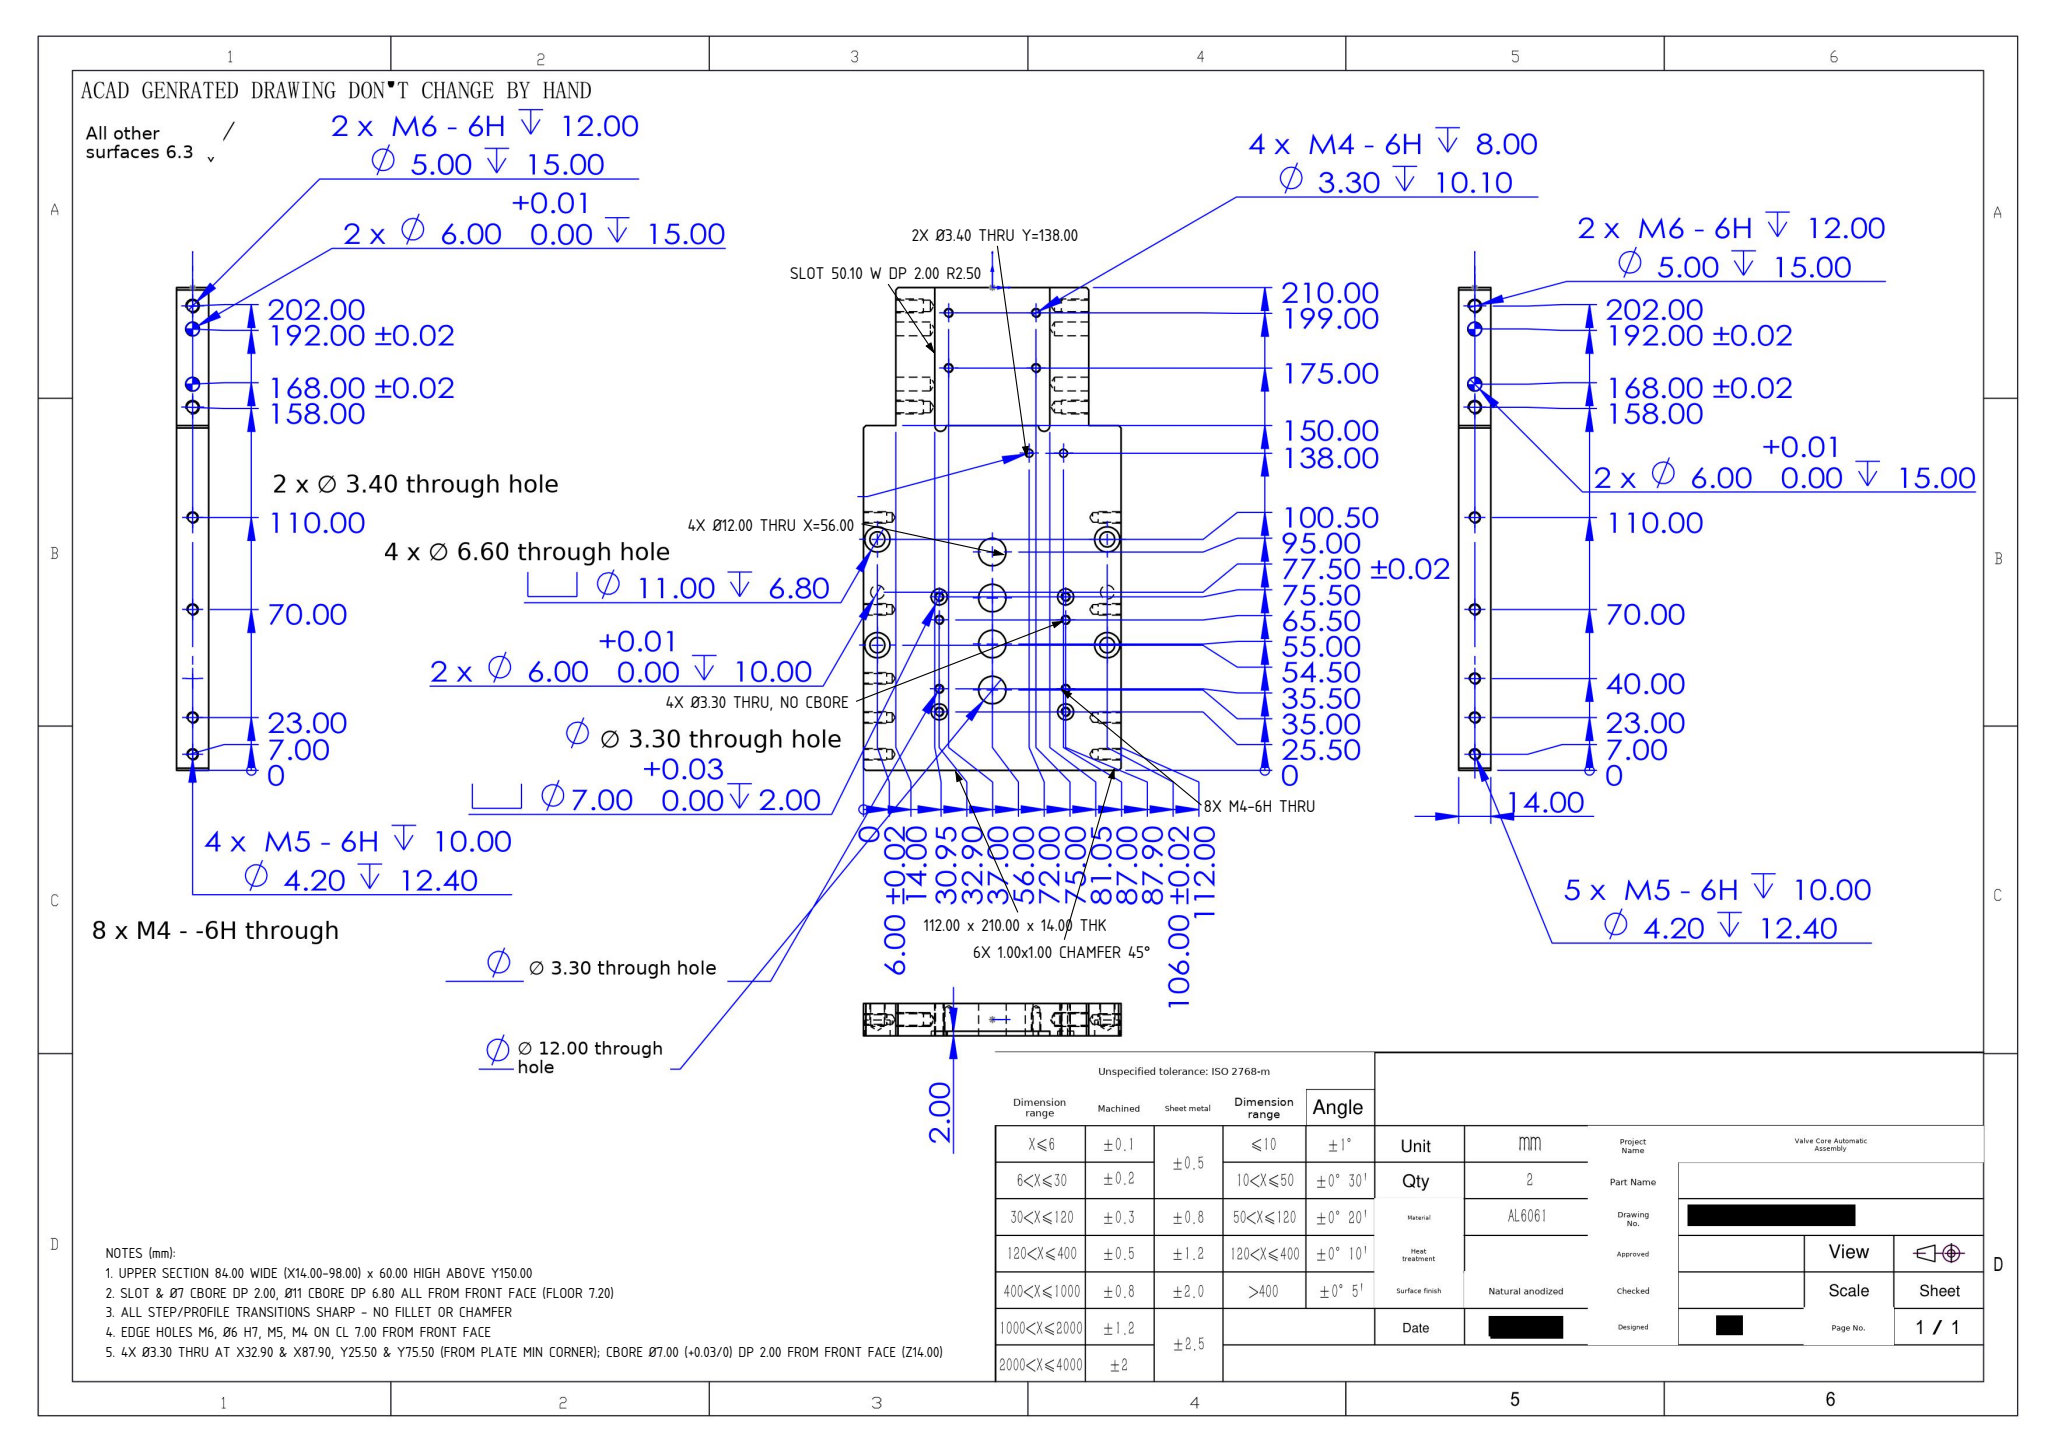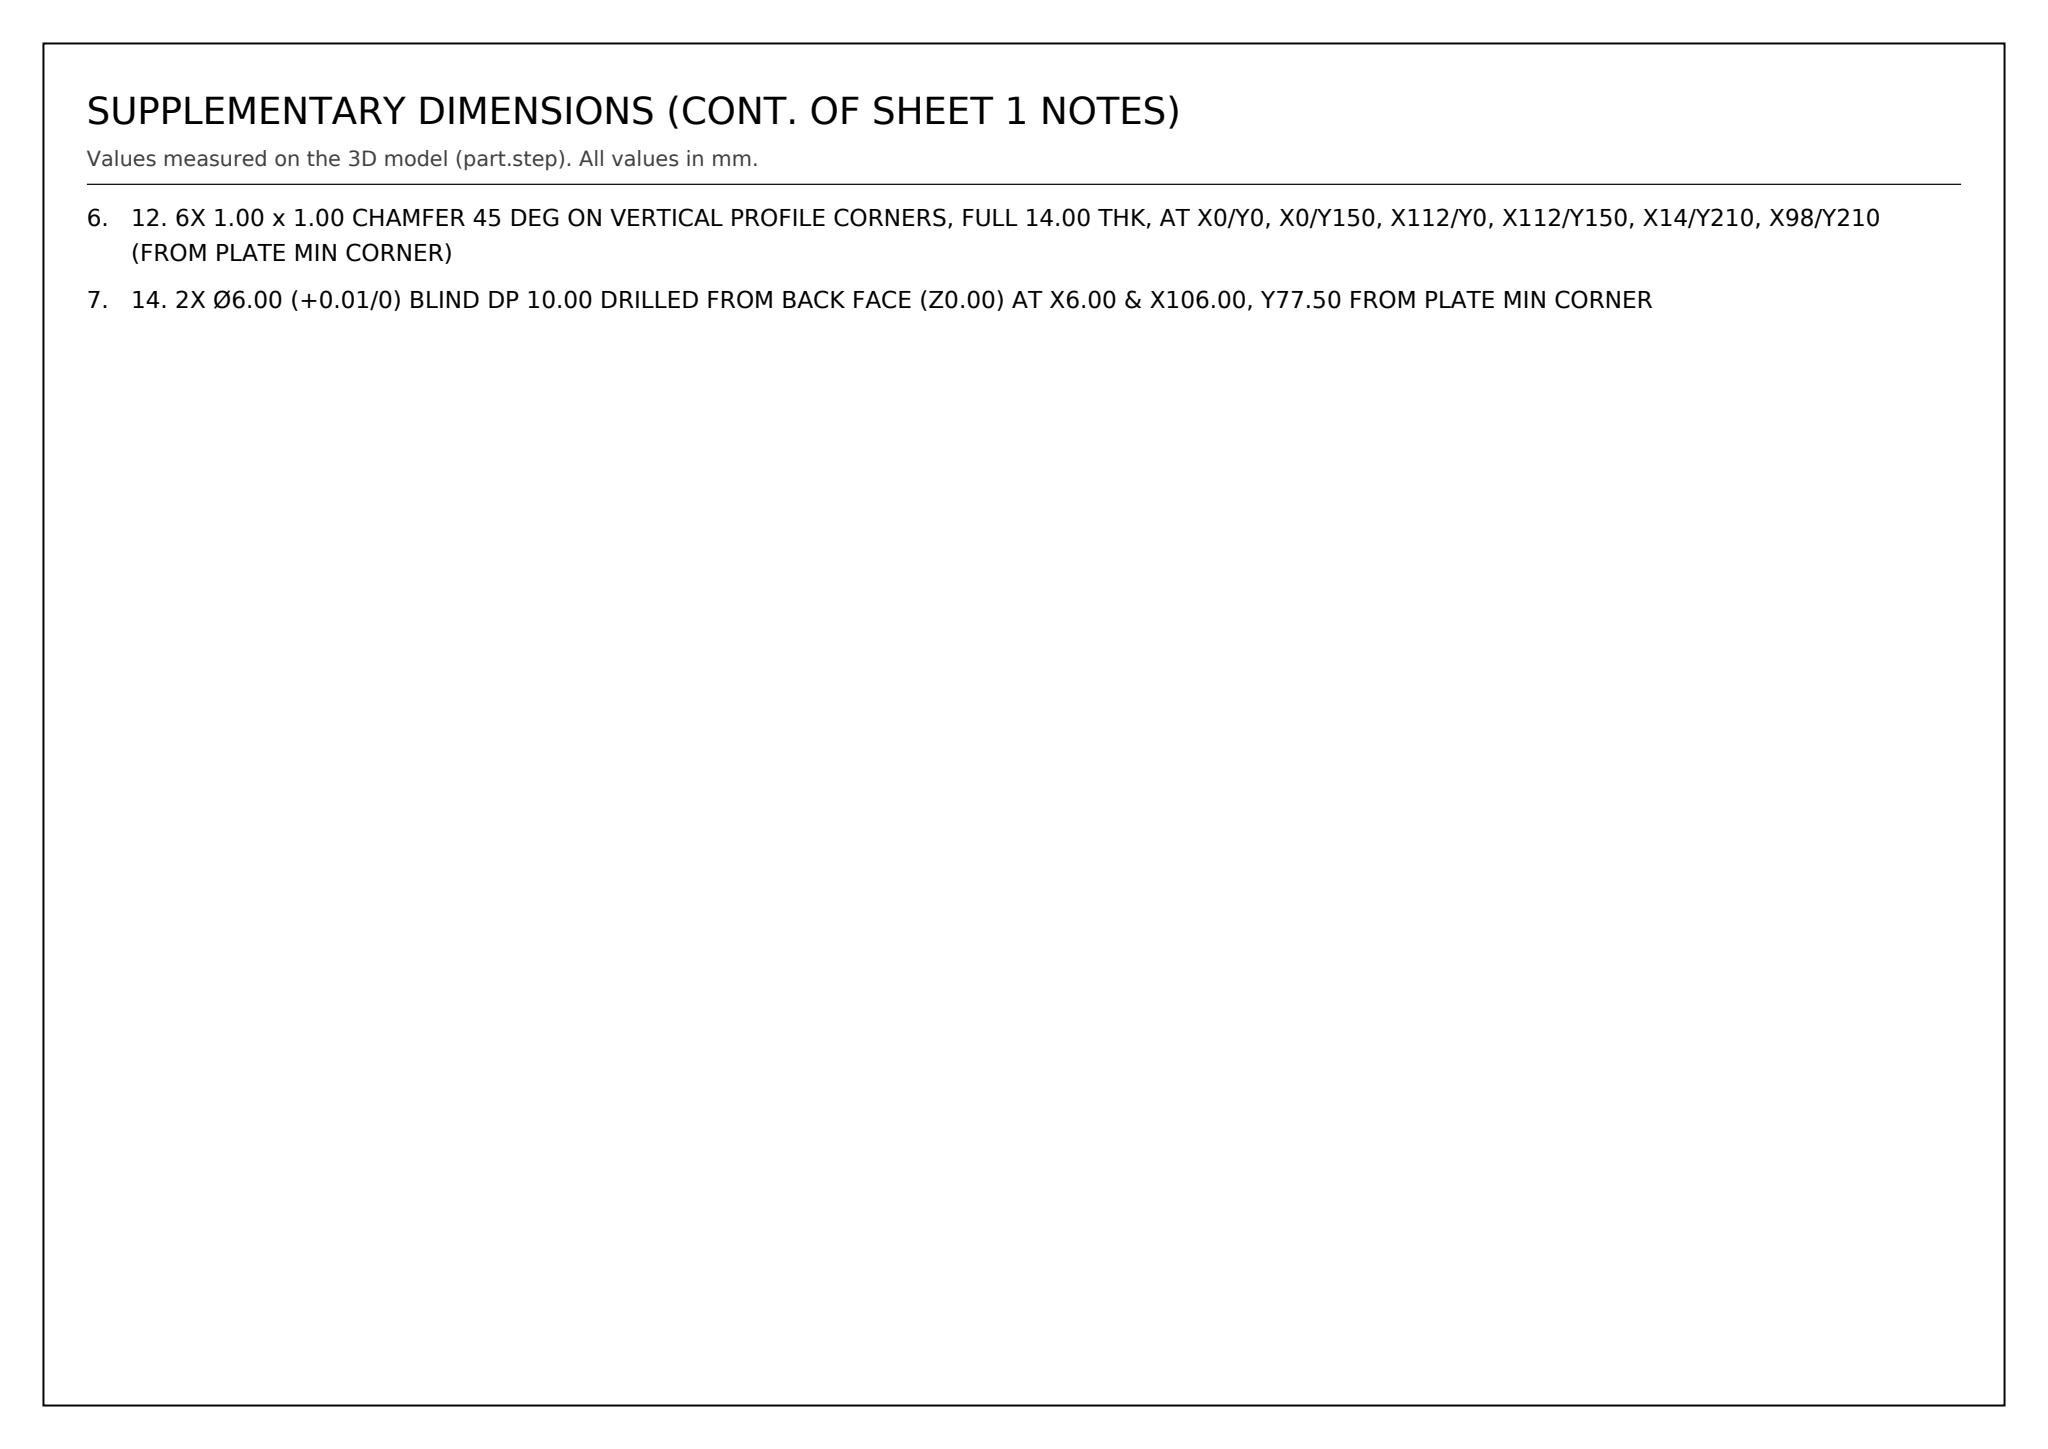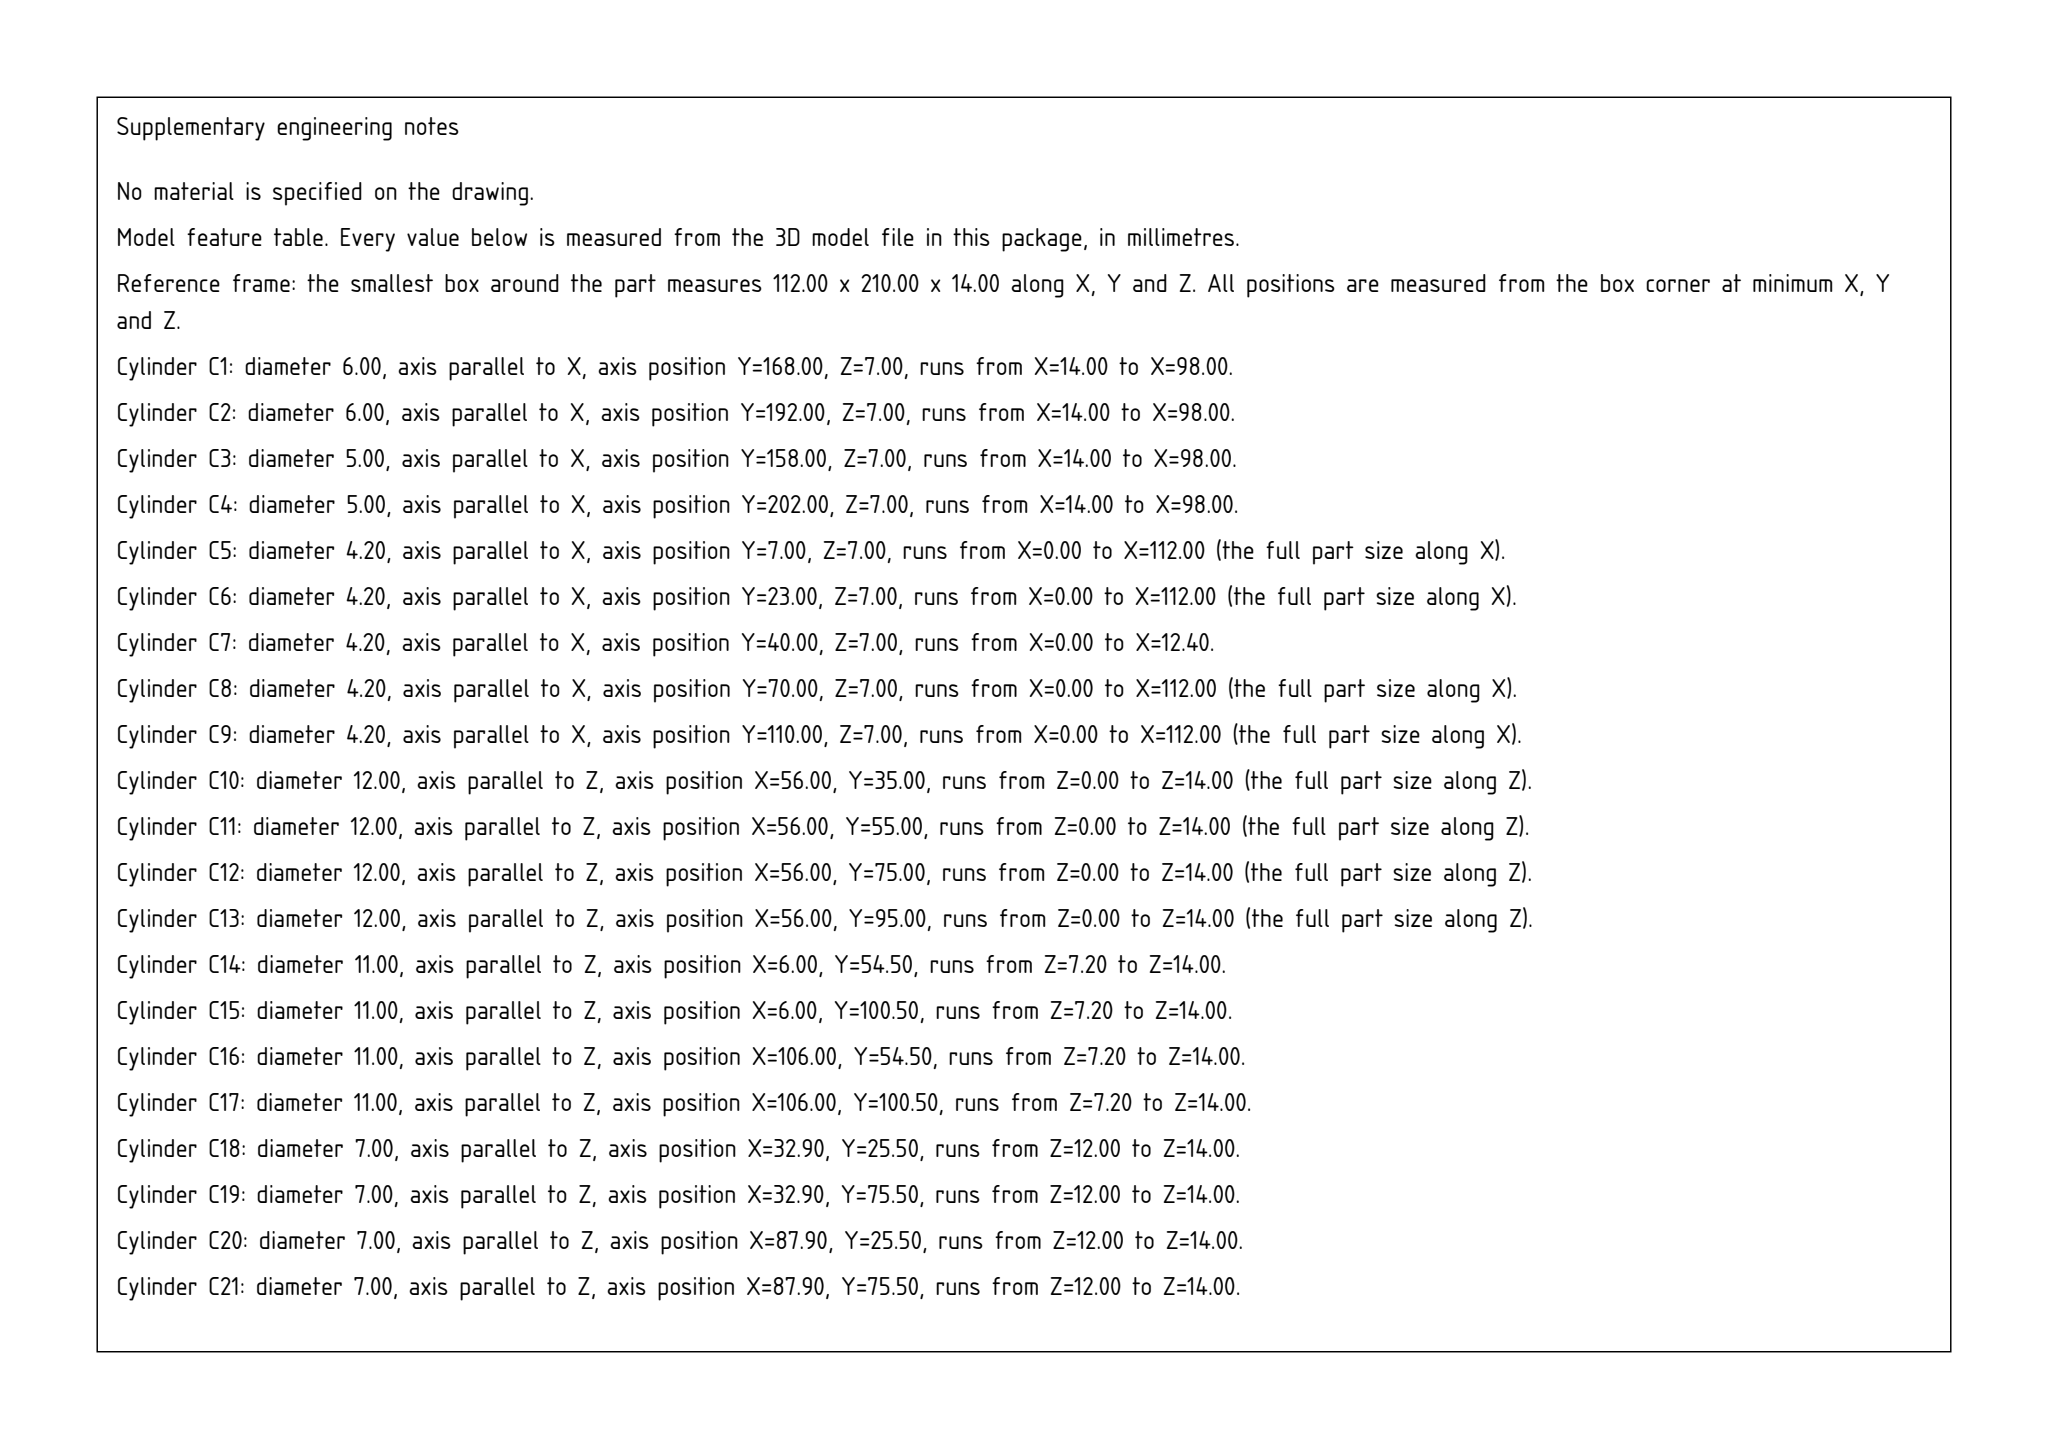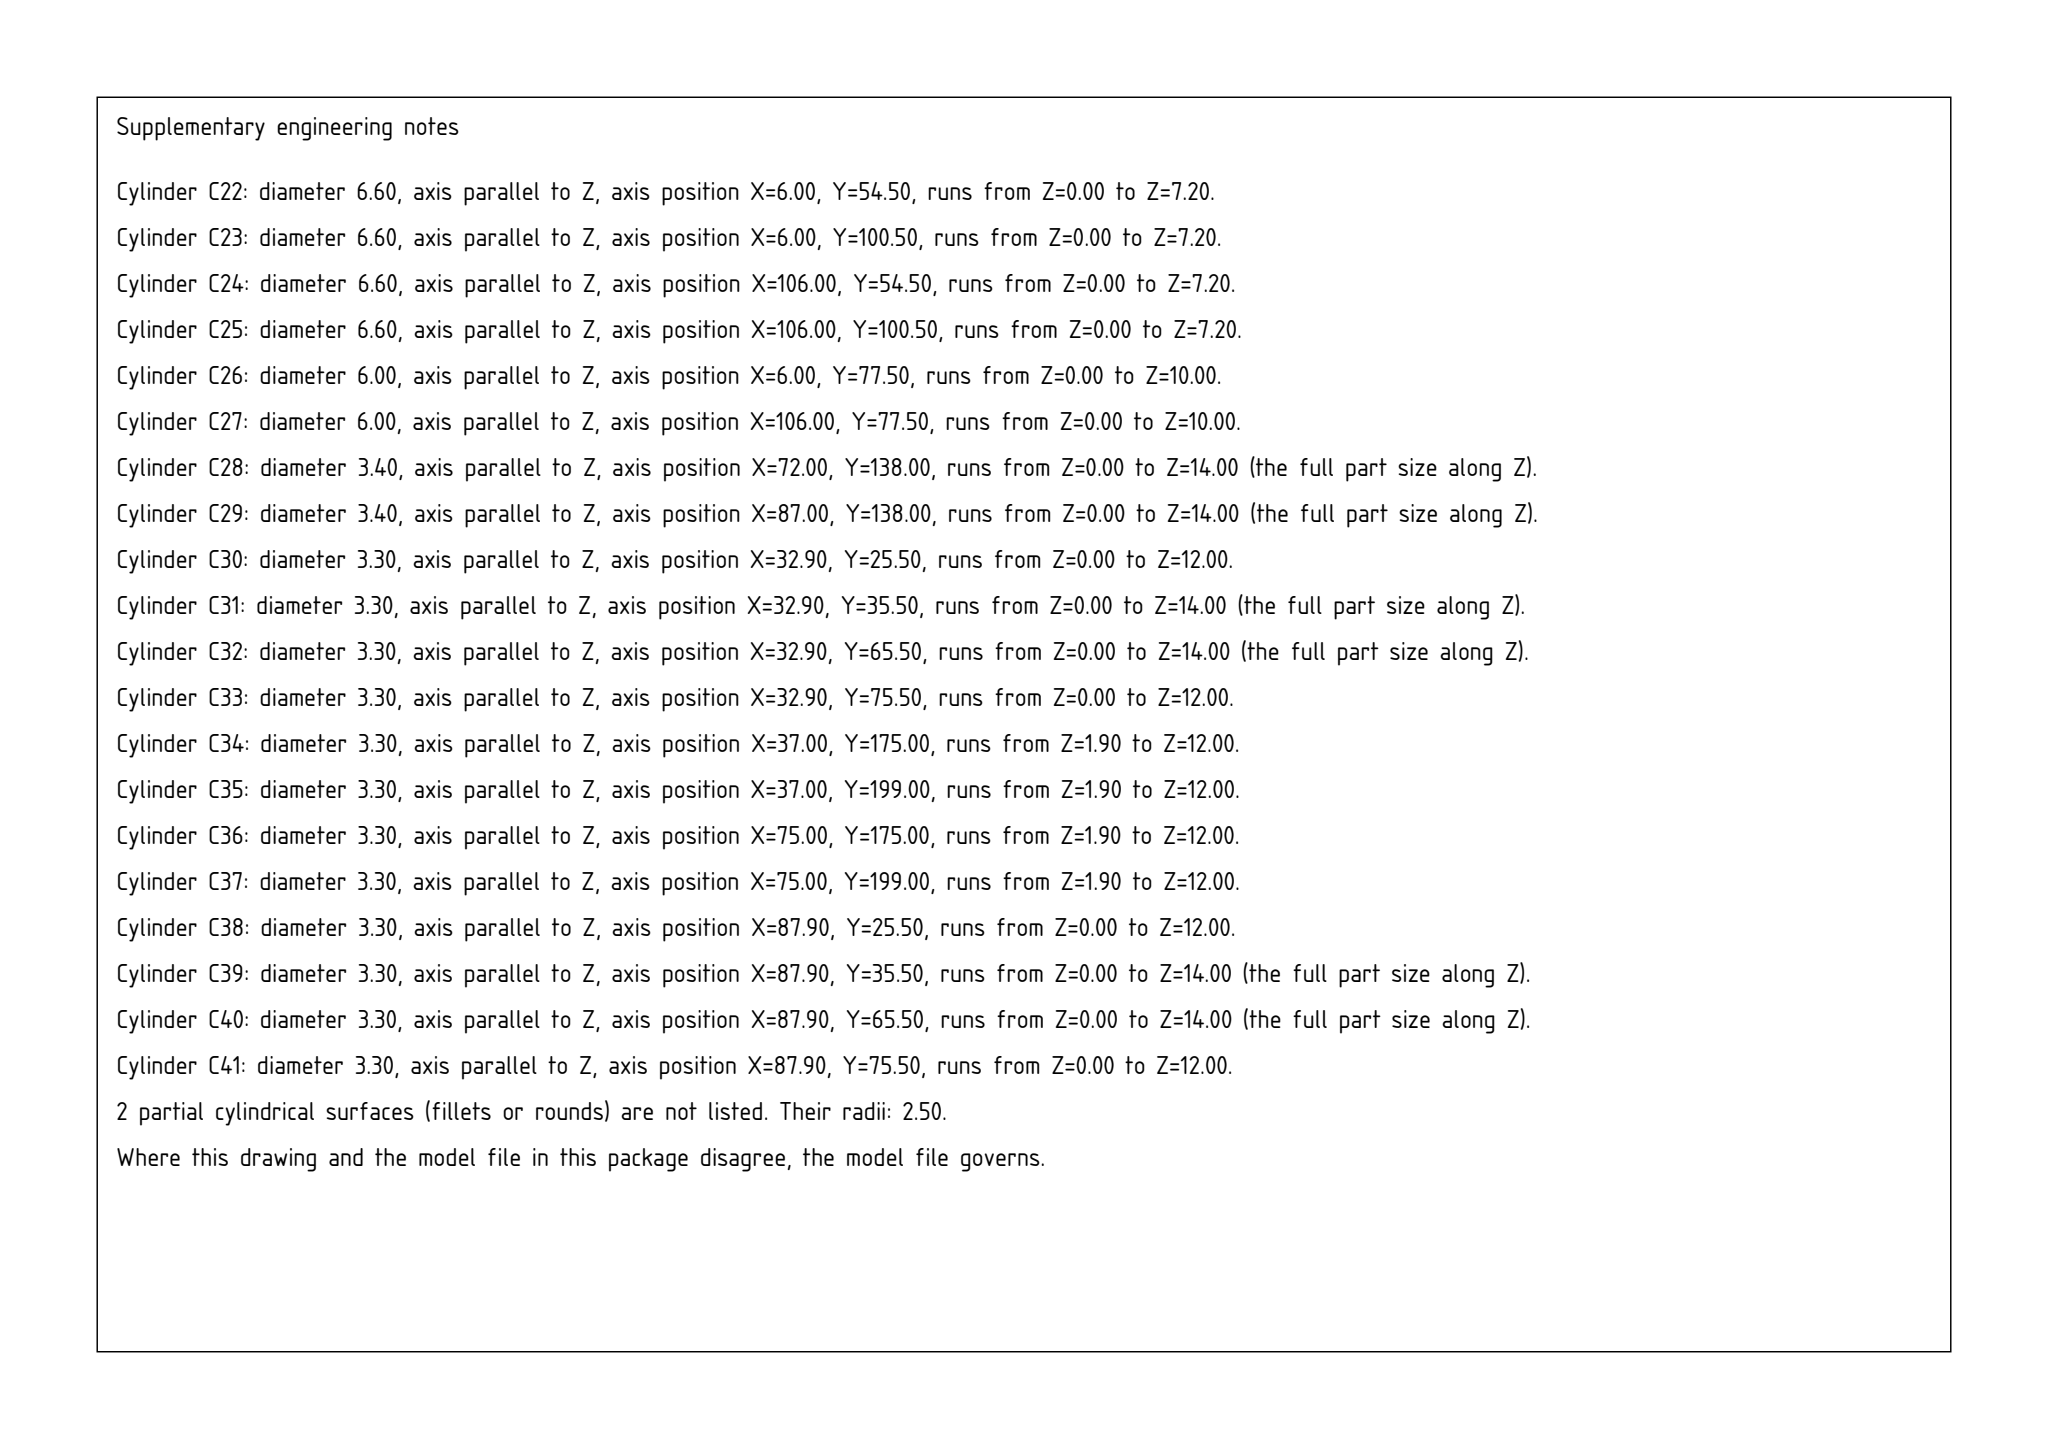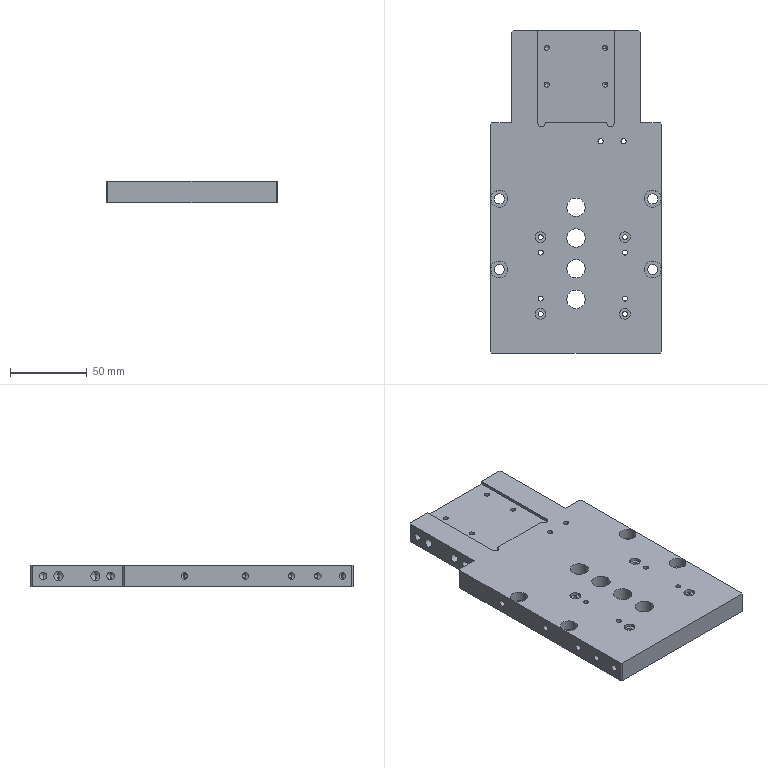Part | SolidWorks | mm | material AL6061 | 1 solid | 174 faces | box 112 x 210 x 14 mm | volume 282775 mm3 | cylinder 100 | cone 46 | plane 28 | commonest cylinder face diameters 3.3 x24 4.2 x18 6 x12 5 x10 7 x8 11 x8 6.6 x8 12 x8
Drawing notes:
PLATE 112.00 x 210.00 x 14.00 THK; UNIFORM, NO STEPS IN Z | from the solid: bbox 112x210, bbox_z=14.0; only full z faces at 0.0 and 14.0
UPPER SECTION 84.00 WIDE (X14.00-98.00) x 60.00 HIGH ABOVE Y150.00 | from the solid: X planes 14.0 & 98.0 bound upper section; Y 150.0 step to 210.0 top
SLOT 50.10 WIDE (X30.95-81.05) OPEN AT TOP, DP 2.00, END Y150.00, R2.50 CNRS | from the solid: X planes 30.95/81.05; floor z=12.0 (14.0-2.0); open face at y=210; Ø5 z-cyls at (33.45,150) & (78.55,150) len 2.0; 3 faces at y=150
SLOT & Ø7 CBORE DP 2.00, Ø11 CBORE DP 6.80 ALL FROM FRONT FACE (FLOOR 7.20) | from the solid: z planes 12.0 (slot floor + 4x Ø7 cbore) and 7.2 (4x Ø11 cbore = 14.0-6.8)
ALL STEP/PROFILE TRANSITIONS SHARP - NO FILLET OR CHAMFER | from the solid: fillet_radii empty; no cones except 118° drill points
4 x Ø12.00 THRU AT X56.00; Y35.00, 55.00, 75.00, 95.00 | from the solid: Ø12 z-cyls len 14.0 at (56,35), (56,55), (56,75), (56,95)
2 x Ø3.40 THRU AT Y138.00; X72.00 & 87.00 | from the solid: Ø3.4 z-cyls at (72.0,138.0) and (87.0,138.0), length 14.0 = full thk
8 x M4-6H THRU AT X32.90 & 87.90; Y25.50, 35.50, 65.50, 75.50 | from the solid: Ø3.30 z-holes at x=32.9 & 87.9, y=25.5/35.5/65.5/75.5, thru 14.0 or 12.0 under Ø7 CBORE
EDGE HOLES M6, Ø6 H7, M5, M4 ON CL 7.00 FROM FRONT FACE | from the solid: x-axis cylinders Ø4.2/5.0/6.0 all at z=7.0 of 14.0 thk plate
4X Ø3.30 THRU AT X32.90 & X87.90, Y25.50 & Y75.50 (FROM PLATE MIN CORNER); CBORE Ø7.00 (+0.03/0) DP 2.00 FROM FRONT FACE (Z14.00) | from the solid: cylinders: Ø3.3 z-holes at (32.9,25.5),(32.9,75.5),(87.9,25.5),(87.9,75.5) from 0.0 to 12.0, each with Ø7.0 z-bore from 12.0 to 14.0
4X Ø3.30 THRU (NO CBORE) AT X32.90 & X87.90, Y35.50 & Y65.50 FROM PLATE MIN CORNER | from the solid: cylinders: Ø3.3 z-holes at (32.9,35.5),(32.9,65.5),(87.9,35.5),(87.9,65.5) from 0.0 to 14.0
12. 6X 1.00 x 1.00 CHAMFER 45 DEG ON VERTICAL PROFILE CORNERS, FULL 14.00 THK, AT X0/Y0, X0/Y150, X112/Y0, X112/Y150, X14/Y210, X98/Y210 (FROM PLATE MIN CORNER) | from the solid: inclined_planes: six 45/45/90 faces, size [1.0,1.0,14.0] at bbox_from [0,0,0], [0,149,0], [111,0,0], [111,149,0], [14,209,0], [97,209,0]
13. NOTE 5 APPLIES EXCEPT FOR THE 6X 1.00 x 1.00 CORNER CHAMFERS OF NOTE 12; ALL OTHER STEP/PROFILE TRANSITIONS SHARP | from the solid: inclined_planes list contains only the six 1.00 x 1.00 x 14.00 45 deg corner faces; tori list empty (no fillets)
14. 2X Ø6.00 (+0.01/0) BLIND DP 10.00 DRILLED FROM BACK FACE (Z0.00) AT X6.00 & X106.00, Y77.50 FROM PLATE MIN CORNER | from the solid: cylinders: dia 6.0 axis z at [6.0,77.5] and [106.0,77.5], from 0.0 to 10.0 (plate Z extent 0-14, front face Z14.00)
build123d program:
from build123d import *

# Parameters (mm, degrees)
BOSS_EXTRUDE1_DEPTH                                = 7
SKETCH2_W                                          = 50.1
SKETCH2_H                                          = 60
CUT_EXTRUDE1_DEPTH                                 = 2
SKETCH4_W                                          = 54
SKETCH4_H                                          = 150
CUT_EXTRUDE5_DEPTH                                 = 238.478
SKETCH5_W                                          = 14
SKETCH5_H                                          = 60
CUT_EXTRUDE6_DEPTH                                 = 218.789
M3_CLEARANCE_HOLE1_D                               = 3.4
SKETCH8_R                                          = 6
CUT_EXTRUDE7_DEPTH                                 = 218.789
SKETCH9_R                                          = 2.5
CUT_EXTRUDE8_DEPTH                                 = 2
HOLE_SIZE_ACCORDING_TO_TYPE_1_OF_HEXAG_D           = 6.6
HOLE_SIZE_ACCORDING_TO_TYPE_1_OF_HEXAG_CBORE_D     = 11
HOLE_SIZE_ACCORDING_TO_TYPE_1_OF_HEXAG_CBORE_DEPTH = 6.8
SIZE_MM_DOWEL_PIN_HOLE1_D                          = 6
SIZE_MM_DOWEL_PIN_HOLE1_DEPTH                      = 10
SIZE_MM_DOWEL_PIN_HOLE1_TIP                        = 1.803
M6_TAPPED_HOLE1_D                                  = 5
M6_TAPPED_HOLE1_DEPTH                              = 15
M6_TAPPED_HOLE1_TIP                                = 1.502
M6_TAPPED_HOLE2_D                                  = 5
M6_TAPPED_HOLE2_DEPTH                              = 15
M6_TAPPED_HOLE2_TIP                                = 1.502
SIZE_MM_DOWEL_PIN_HOLE2_D                          = 6
SIZE_MM_DOWEL_PIN_HOLE2_DEPTH                      = 15
SIZE_MM_DOWEL_PIN_HOLE2_TIP                        = 1.803
SIZE_MM_DOWEL_PIN_HOLE3_D                          = 6
SIZE_MM_DOWEL_PIN_HOLE3_DEPTH                      = 15
SIZE_MM_DOWEL_PIN_HOLE3_TIP                        = 1.803
M4_TAPPED_HOLE1_D                                  = 3.3
SKETCH24_R                                         = 3.5
CUT_EXTRUDE9_DEPTH                                 = 2
M5_TAPPED_HOLE1_D                                  = 4.2
M5_TAPPED_HOLE1_DEPTH                              = 12.4
M5_TAPPED_HOLE1_TIP                                = 1.262
M5_TAPPED_HOLE2_D                                  = 4.2
M5_TAPPED_HOLE2_DEPTH                              = 12.4
M5_TAPPED_HOLE2_TIP                                = 1.262
M4_TAPPED_HOLE2_D                                  = 3.3
M4_TAPPED_HOLE2_DEPTH                              = 10.1
M4_TAPPED_HOLE2_TIP                                = 0.9914
CHAMFER1_SIZE                                      = 1


with BuildPart() as part:
    # Sketch1 → Boss-Extrude1 (new, symmetric)
    with BuildSketch(Plane.XY):
        Polygon((56, 0), (-56, 0), (-56, -60), (-110, -60), (-110, -210), (110, -210), (110, -60), (56, -60), align=None)
    extrude(amount=BOSS_EXTRUDE1_DEPTH, both=True)

    # Sketch2 → Cut-Extrude1 (cut)
    with BuildSketch(Plane.XY.offset(7)):
        with Locations((0, -30)):
            Rectangle(SKETCH2_W, SKETCH2_H)
    extrude(amount=-CUT_EXTRUDE1_DEPTH, mode=Mode.SUBTRACT)

    # Sketch4 → Cut-Extrude5 (cut, through all)
    with BuildSketch(Plane.XY.offset(7)):
        with Locations((-83, -135)):
            Rectangle(SKETCH4_W, SKETCH4_H)
        with Locations((83, -135)):
            Rectangle(SKETCH4_W, SKETCH4_H)
    extrude(amount=-CUT_EXTRUDE5_DEPTH, mode=Mode.SUBTRACT)

    # Sketch5 → Cut-Extrude6 (cut, through all)
    with BuildSketch(Plane.XY.offset(7)):
        with Locations((49, -30)):
            Rectangle(SKETCH5_W, SKETCH5_H)
        with Locations((-49, -30)):
            Rectangle(SKETCH5_W, SKETCH5_H)
    extrude(amount=-CUT_EXTRUDE6_DEPTH, mode=Mode.SUBTRACT)

    # M3 Clearance Hole1 (through all)
    with Locations(Plane(origin=(0, 0, -7), x_dir=(-1, 0, 0), z_dir=(0, 0, -1))):
        with Locations((-16, -72), (-31, -72)):
            Hole(M3_CLEARANCE_HOLE1_D / 2)

    # Sketch8 → Cut-Extrude7 (cut, through all)
    with BuildSketch(Plane(origin=(0, 0, -7), x_dir=(-1, 0, 0), z_dir=(0, 0, -1))):
        with Locations((0, -115)):
            Circle(SKETCH8_R)
        with Locations((0, -155)):
            Circle(SKETCH8_R)
        with Locations((0, -135)):
            Circle(SKETCH8_R)
        with Locations((0, -175)):
            Circle(SKETCH8_R)
    extrude(amount=-CUT_EXTRUDE7_DEPTH, mode=Mode.SUBTRACT)

    # Sketch9 → Cut-Extrude8 (cut)
    with BuildSketch(Plane.XY.offset(7)):
        with Locations((-22.55, -60)):
            Circle(SKETCH9_R)
        with Locations((22.55, -60)):
            Circle(SKETCH9_R)
    extrude(amount=-CUT_EXTRUDE8_DEPTH, mode=Mode.SUBTRACT)

    # Hole Size _According to_ Type 1 of Hexag (through all)
    with Locations(Plane.XY.offset(7)):
        with Locations((50, -109.5), (-50, -109.5), (50, -155.5), (-50, -155.5)):
            CounterBoreHole(HOLE_SIZE_ACCORDING_TO_TYPE_1_OF_HEXAG_D / 2, HOLE_SIZE_ACCORDING_TO_TYPE_1_OF_HEXAG_CBORE_D / 2, HOLE_SIZE_ACCORDING_TO_TYPE_1_OF_HEXAG_CBORE_DEPTH)

    # Size mm Dowel Pin Hole1
    with Locations(Plane(origin=(0, 0, -7), x_dir=(-1, 0, 0), z_dir=(0, 0, -1))):
        with Locations((-50, -132.5), (50, -132.5)):
            Hole(SIZE_MM_DOWEL_PIN_HOLE1_D / 2, depth=SIZE_MM_DOWEL_PIN_HOLE1_DEPTH)
            with Locations((0, 0, -(SIZE_MM_DOWEL_PIN_HOLE1_DEPTH + SIZE_MM_DOWEL_PIN_HOLE1_TIP / 2))):  # 118° drill point
                Cone(0, SIZE_MM_DOWEL_PIN_HOLE1_D / 2, SIZE_MM_DOWEL_PIN_HOLE1_TIP, mode=Mode.SUBTRACT)

    # M6 Tapped Hole1
    with Locations(Plane(origin=(42, 0, 0), x_dir=(0, 0, -1), z_dir=(1, 0, 0))):
        with Locations((0, -52), (0, -8)):
            Hole(M6_TAPPED_HOLE1_D / 2, depth=M6_TAPPED_HOLE1_DEPTH)
            with Locations((0, 0, -(M6_TAPPED_HOLE1_DEPTH + M6_TAPPED_HOLE1_TIP / 2))):  # 118° drill point
                Cone(0, M6_TAPPED_HOLE1_D / 2, M6_TAPPED_HOLE1_TIP, mode=Mode.SUBTRACT)

    # M6 Tapped Hole2
    with Locations(Plane.ZY.offset(42)):
        with Locations((0, -8), (0, -52)):
            Hole(M6_TAPPED_HOLE2_D / 2, depth=M6_TAPPED_HOLE2_DEPTH)
            with Locations((0, 0, -(M6_TAPPED_HOLE2_DEPTH + M6_TAPPED_HOLE2_TIP / 2))):  # 118° drill point
                Cone(0, M6_TAPPED_HOLE2_D / 2, M6_TAPPED_HOLE2_TIP, mode=Mode.SUBTRACT)

    # Size mm Dowel Pin Hole2
    with Locations(Plane.ZY.offset(42)):
        with Locations((0, -42), (0, -18)):
            Hole(SIZE_MM_DOWEL_PIN_HOLE2_D / 2, depth=SIZE_MM_DOWEL_PIN_HOLE2_DEPTH)
            with Locations((0, 0, -(SIZE_MM_DOWEL_PIN_HOLE2_DEPTH + SIZE_MM_DOWEL_PIN_HOLE2_TIP / 2))):  # 118° drill point
                Cone(0, SIZE_MM_DOWEL_PIN_HOLE2_D / 2, SIZE_MM_DOWEL_PIN_HOLE2_TIP, mode=Mode.SUBTRACT)

    # Size mm Dowel Pin Hole3
    with Locations(Plane(origin=(42, 0, 0), x_dir=(0, 0, -1), z_dir=(1, 0, 0))):
        with Locations((0, -18), (0, -42)):
            Hole(SIZE_MM_DOWEL_PIN_HOLE3_D / 2, depth=SIZE_MM_DOWEL_PIN_HOLE3_DEPTH)
            with Locations((0, 0, -(SIZE_MM_DOWEL_PIN_HOLE3_DEPTH + SIZE_MM_DOWEL_PIN_HOLE3_TIP / 2))):  # 118° drill point
                Cone(0, SIZE_MM_DOWEL_PIN_HOLE3_D / 2, SIZE_MM_DOWEL_PIN_HOLE3_TIP, mode=Mode.SUBTRACT)

    # M4 Tapped Hole1 (through all)
    with Locations(Plane.XY.offset(7)):
        with Locations((-23.1, -184.5), (31.9, -184.5), (31.9, -174.5), (31.9, -144.5), (31.9, -134.5), (-23.1, -134.5), (-23.1, -144.5), (-23.1, -174.5)):
            Hole(M4_TAPPED_HOLE1_D / 2)

    # Sketch24 → Cut-Extrude9 (cut)
    with BuildSketch(Plane.XY.offset(7)):
        with Locations((31.9, -134.5)):
            Circle(SKETCH24_R)
        with Locations((-23.1, -134.5)):
            Circle(SKETCH24_R)
        with Locations((-23.1, -184.5)):
            Circle(SKETCH24_R)
        with Locations((31.9, -184.5)):
            Circle(SKETCH24_R)
    extrude(amount=-CUT_EXTRUDE9_DEPTH, mode=Mode.SUBTRACT)

    # M5 Tapped Hole1
    with Locations(Plane.ZY.offset(56)):
        with Locations((0, -170), (0, -203), (0, -187), (0, -100), (0, -140)):
            Hole(M5_TAPPED_HOLE1_D / 2, depth=M5_TAPPED_HOLE1_DEPTH)
            with Locations((0, 0, -(M5_TAPPED_HOLE1_DEPTH + M5_TAPPED_HOLE1_TIP / 2))):  # 118° drill point
                Cone(0, M5_TAPPED_HOLE1_D / 2, M5_TAPPED_HOLE1_TIP, mode=Mode.SUBTRACT)

    # M5 Tapped Hole2
    with Locations(Plane(origin=(56, 0, 0), x_dir=(0, 0, -1), z_dir=(1, 0, 0))):
        with Locations((0, -187), (0, -203), (0, -100), (0, -140)):
            Hole(M5_TAPPED_HOLE2_D / 2, depth=M5_TAPPED_HOLE2_DEPTH)
            with Locations((0, 0, -(M5_TAPPED_HOLE2_DEPTH + M5_TAPPED_HOLE2_TIP / 2))):  # 118° drill point
                Cone(0, M5_TAPPED_HOLE2_D / 2, M5_TAPPED_HOLE2_TIP, mode=Mode.SUBTRACT)

    # M4 Tapped Hole2
    with Locations(Plane.XY.offset(5)):
        with Locations((19, -11), (-19, -11), (19, -35), (-19, -35)):
            Hole(M4_TAPPED_HOLE2_D / 2, depth=M4_TAPPED_HOLE2_DEPTH)
            with Locations((0, 0, -(M4_TAPPED_HOLE2_DEPTH + M4_TAPPED_HOLE2_TIP / 2))):  # 118° drill point
                Cone(0, M4_TAPPED_HOLE2_D / 2, M4_TAPPED_HOLE2_TIP, mode=Mode.SUBTRACT)

    # Chamfer1
    chamfer1_edges = [part.edges().sort_by_distance(p)[0] for p in [
        (42, 0, 0),
        (56, -60, 0),
        (-56, -210, 0),
        (56, -210, 0),
        (-56, -60, 0),
        (-42, 0, 0),
    ]]
    chamfer(chamfer1_edges, length=CHAMFER1_SIZE)


solid = part.part